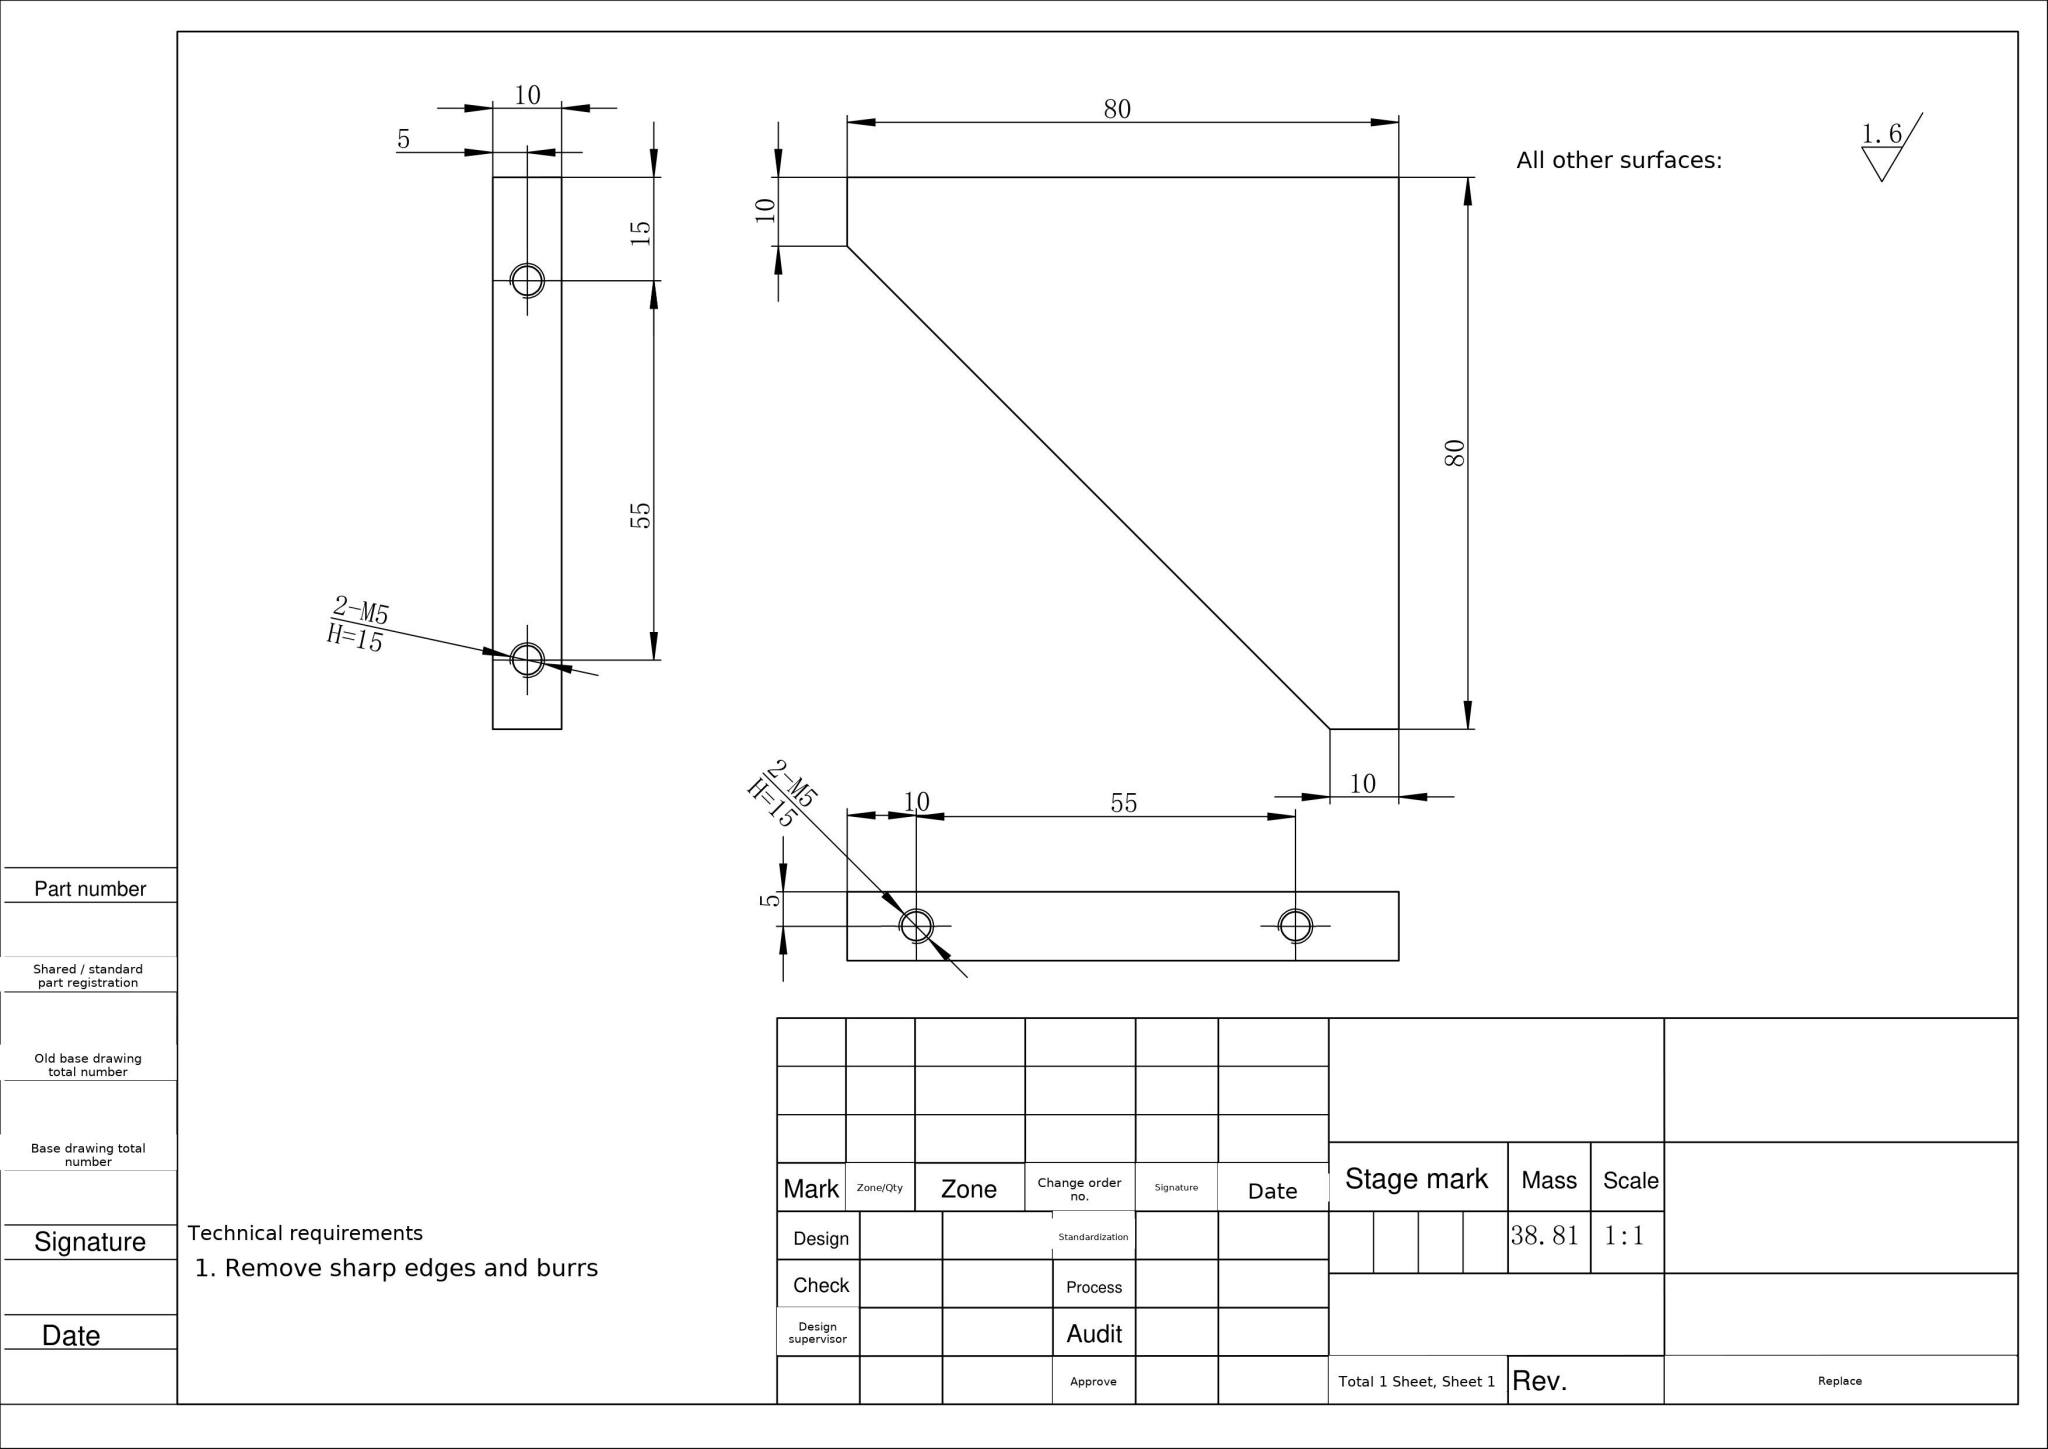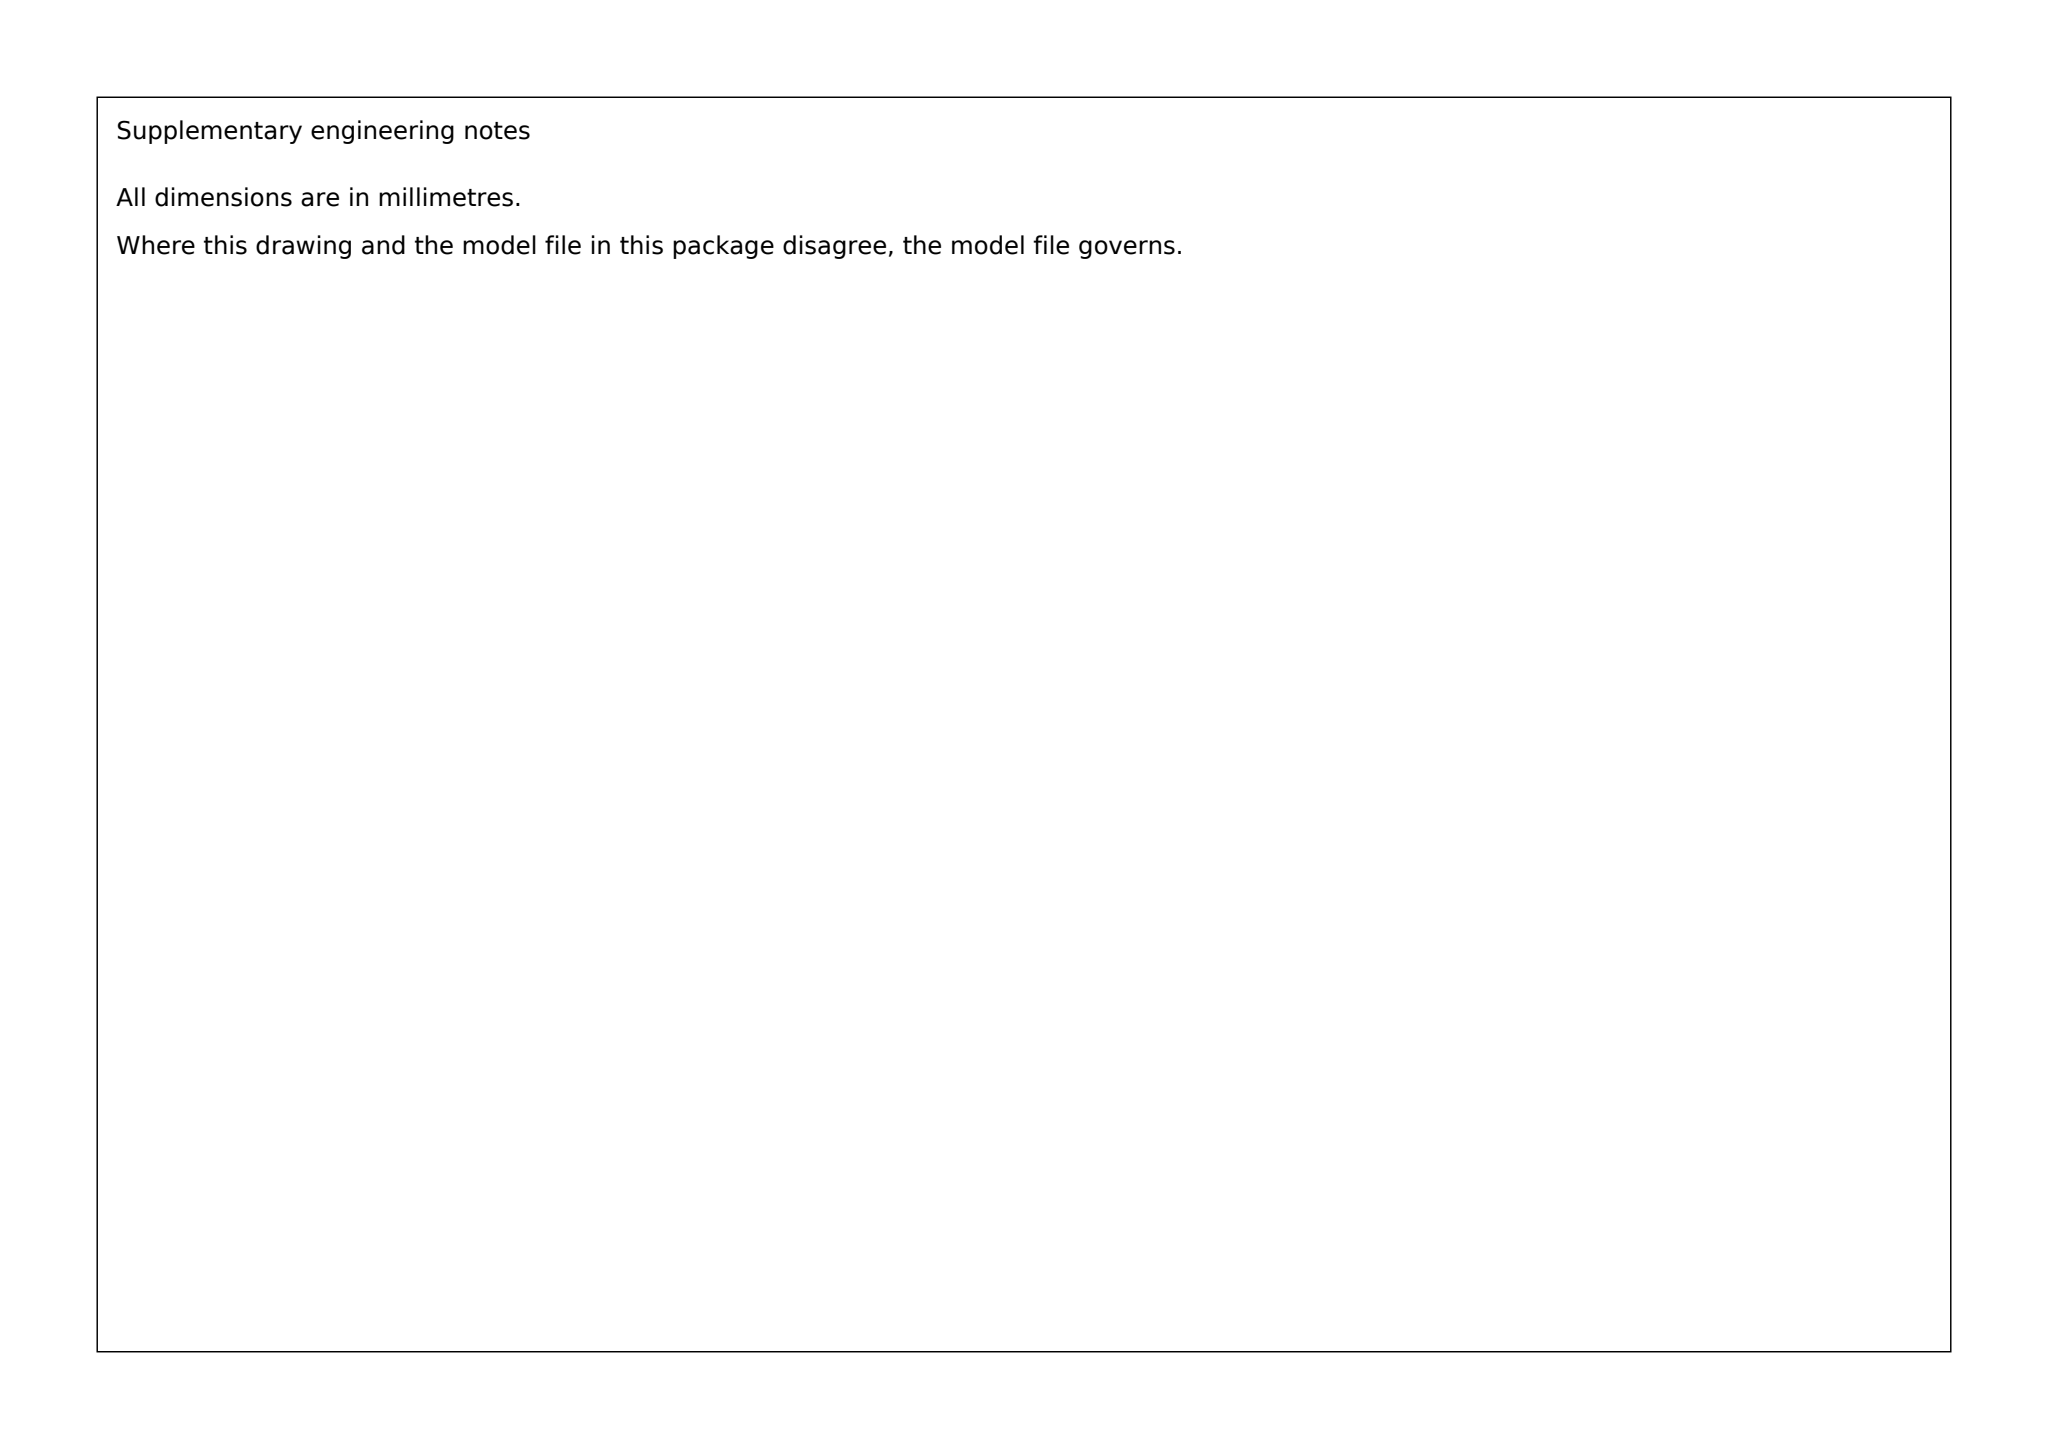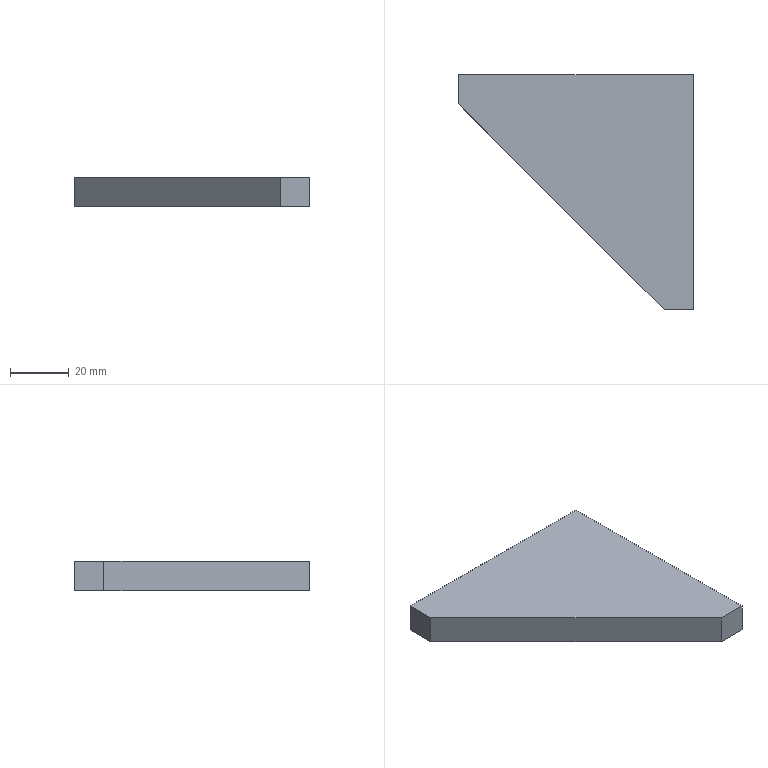Part | SolidWorks | mm | 1 solid | 23 faces | box 80 x 80 x 10 mm | volume 38812 mm3 | cylinder 8 | cone 8 | plane 7 | commonest cylinder face diameters 4.2 x8
build123d program:
from build123d import *

# Parameters (mm, degrees)
BOSS_EXTRUDE1_DEPTH   = 10
M5_TAPPED_HOLE1_D     = 4.2
M5_TAPPED_HOLE1_DEPTH = 12
M5_TAPPED_HOLE1_TIP   = 1.262
M5_TAPPED_HOLE2_D     = 4.2
M5_TAPPED_HOLE2_DEPTH = 12
M5_TAPPED_HOLE2_TIP   = 1.262


with BuildPart() as part:
    # Sketch1 → Boss-Extrude1 (new body)
    with BuildSketch(Plane.XY):
        Polygon((571.382, 0), (571.382, -80), (561.382, -80), (491.382, -10), (491.382, 0), align=None)
    extrude(amount=-BOSS_EXTRUDE1_DEPTH)

    # M5 Tapped Hole1
    with Locations(Plane(origin=(0, 0, 0), x_dir=(1, 0, 0), z_dir=(0, 1, 0))):
        with Locations((556.382, 5), (501.382, 5)):
            Hole(M5_TAPPED_HOLE1_D / 2, depth=M5_TAPPED_HOLE1_DEPTH)
            with Locations((0, 0, -(M5_TAPPED_HOLE1_DEPTH + M5_TAPPED_HOLE1_TIP / 2))):  # 118° drill point
                Cone(0, M5_TAPPED_HOLE1_D / 2, M5_TAPPED_HOLE1_TIP, mode=Mode.SUBTRACT)

    # M5 Tapped Hole2
    with Locations(Plane(origin=(571.382, 0, 0), x_dir=(0, 0, -1), z_dir=(1, 0, 0))):
        with Locations((5, -70), (5, -15)):
            Hole(M5_TAPPED_HOLE2_D / 2, depth=M5_TAPPED_HOLE2_DEPTH)
            with Locations((0, 0, -(M5_TAPPED_HOLE2_DEPTH + M5_TAPPED_HOLE2_TIP / 2))):  # 118° drill point
                Cone(0, M5_TAPPED_HOLE2_D / 2, M5_TAPPED_HOLE2_TIP, mode=Mode.SUBTRACT)


solid = part.part
STEP:
#1=CARTESIAN_POINT('',(559.382,-15.,-2.9));
#2=VERTEX_POINT('',#1);
#3=CARTESIAN_POINT('',(559.382,-15.,-7.1));
#4=VERTEX_POINT('',#3);
#5=CARTESIAN_POINT('',(559.382,-15.,-5.));
#6=DIRECTION('',(1.,0.,0.));
#7=DIRECTION('',(0.,0.,-1.));
#8=AXIS2_PLACEMENT_3D('',#5,#6,#7);
#9=CIRCLE('',#8,2.1);
#10=EDGE_CURVE('',#2,#4,#9,.T.);
#11=ORIENTED_EDGE('',*,*,#10,.F.);
#12=CARTESIAN_POINT('',(571.382,-15.,-2.9));
#13=VERTEX_POINT('',#12);
#14=CARTESIAN_POINT('',(571.382,-15.,-2.9));
#15=DIRECTION('',(1.,0.,0.));
#16=VECTOR('',#15,1000.);
#17=LINE('',#14,#16);
#18=EDGE_CURVE('',#2,#13,#17,.T.);
#19=ORIENTED_EDGE('',*,*,#18,.T.);
#20=CARTESIAN_POINT('',(571.382,-15.,-7.1));
#21=VERTEX_POINT('',#20);
#22=CARTESIAN_POINT('',(571.382,-15.,-5.));
#23=DIRECTION('',(1.,0.,0.));
#24=DIRECTION('',(0.,0.,-1.));
#25=AXIS2_PLACEMENT_3D('',#22,#23,#24);
#26=CIRCLE('',#25,2.1);
#27=EDGE_CURVE('',#13,#21,#26,.T.);
#28=ORIENTED_EDGE('',*,*,#27,.T.);
#29=CARTESIAN_POINT('',(571.382,-15.,-7.1));
#30=DIRECTION('',(1.,0.,0.));
#31=VECTOR('',#30,1000.);
#32=LINE('',#29,#31);
#33=EDGE_CURVE('',#4,#21,#32,.T.);
#34=ORIENTED_EDGE('',*,*,#33,.F.);
#35=EDGE_LOOP('',(#11,#19,#28,#34));
#36=FACE_OUTER_BOUND('',#35,.T.);
#37=CARTESIAN_POINT('',(571.382,-15.,-5.));
#38=DIRECTION('',(1.,0.,0.));
#39=DIRECTION('',(0.,0.,-1.));
#40=AXIS2_PLACEMENT_3D('',#37,#38,#39);
#41=CYLINDRICAL_SURFACE('',#40,2.1);
#42=ADVANCED_FACE('',(#36),#41,.F.);
#43=CARTESIAN_POINT('',(558.12,-15.,-5.));
#44=VERTEX_POINT('',#43);
#45=CARTESIAN_POINT('',(559.382,-15.,-7.1));
#46=DIRECTION('',(0.515,0.,-0.8572));
#47=VECTOR('',#46,1000.);
#48=LINE('',#45,#47);
#49=EDGE_CURVE('',#44,#4,#48,.T.);
#50=ORIENTED_EDGE('',*,*,#49,.F.);
#51=CARTESIAN_POINT('',(559.382,-15.,-2.9));
#52=DIRECTION('',(0.515,0.,0.8572));
#53=VECTOR('',#52,1000.);
#54=LINE('',#51,#53);
#55=EDGE_CURVE('',#44,#2,#54,.T.);
#56=ORIENTED_EDGE('',*,*,#55,.T.);
#57=ORIENTED_EDGE('',*,*,#10,.T.);
#58=EDGE_LOOP('',(#50,#56,#57));
#59=FACE_OUTER_BOUND('',#58,.T.);
#60=CARTESIAN_POINT('',(559.382,-15.,-5.));
#61=DIRECTION('',(1.,0.,0.));
#62=DIRECTION('',(0.,0.,-1.));
#63=AXIS2_PLACEMENT_3D('',#60,#61,#62);
#64=CONICAL_SURFACE('',#63,2.1,1.03);
#65=ADVANCED_FACE('',(#59),#64,.F.);
#66=CARTESIAN_POINT('',(559.382,-70.,-2.9));
#67=VERTEX_POINT('',#66);
#68=CARTESIAN_POINT('',(559.382,-70.,-7.1));
#69=VERTEX_POINT('',#68);
#70=CARTESIAN_POINT('',(559.382,-70.,-5.));
#71=DIRECTION('',(1.,0.,0.));
#72=DIRECTION('',(0.,0.,-1.));
#73=AXIS2_PLACEMENT_3D('',#70,#71,#72);
#74=CIRCLE('',#73,2.1);
#75=EDGE_CURVE('',#67,#69,#74,.T.);
#76=ORIENTED_EDGE('',*,*,#75,.F.);
#77=CARTESIAN_POINT('',(571.382,-70.,-2.9));
#78=VERTEX_POINT('',#77);
#79=CARTESIAN_POINT('',(571.382,-70.,-2.9));
#80=DIRECTION('',(1.,0.,0.));
#81=VECTOR('',#80,1000.);
#82=LINE('',#79,#81);
#83=EDGE_CURVE('',#67,#78,#82,.T.);
#84=ORIENTED_EDGE('',*,*,#83,.T.);
#85=CARTESIAN_POINT('',(571.382,-70.,-7.1));
#86=VERTEX_POINT('',#85);
#87=CARTESIAN_POINT('',(571.382,-70.,-5.));
#88=DIRECTION('',(1.,0.,0.));
#89=DIRECTION('',(0.,0.,-1.));
#90=AXIS2_PLACEMENT_3D('',#87,#88,#89);
#91=CIRCLE('',#90,2.1);
#92=EDGE_CURVE('',#78,#86,#91,.T.);
#93=ORIENTED_EDGE('',*,*,#92,.T.);
#94=CARTESIAN_POINT('',(571.382,-70.,-7.1));
#95=DIRECTION('',(1.,0.,0.));
#96=VECTOR('',#95,1000.);
#97=LINE('',#94,#96);
#98=EDGE_CURVE('',#69,#86,#97,.T.);
#99=ORIENTED_EDGE('',*,*,#98,.F.);
#100=EDGE_LOOP('',(#76,#84,#93,#99));
#101=FACE_OUTER_BOUND('',#100,.T.);
#102=CARTESIAN_POINT('',(571.382,-70.,-5.));
#103=DIRECTION('',(1.,0.,0.));
#104=DIRECTION('',(0.,0.,-1.));
#105=AXIS2_PLACEMENT_3D('',#102,#103,#104);
#106=CYLINDRICAL_SURFACE('',#105,2.1);
#107=ADVANCED_FACE('',(#101),#106,.F.);
#108=CARTESIAN_POINT('',(558.12,-70.,-5.));
#109=VERTEX_POINT('',#108);
#110=CARTESIAN_POINT('',(559.382,-70.,-7.1));
#111=DIRECTION('',(0.515,0.,-0.8572));
#112=VECTOR('',#111,1000.);
#113=LINE('',#110,#112);
#114=EDGE_CURVE('',#109,#69,#113,.T.);
#115=ORIENTED_EDGE('',*,*,#114,.F.);
#116=CARTESIAN_POINT('',(559.382,-70.,-2.9));
#117=DIRECTION('',(0.515,0.,0.8572));
#118=VECTOR('',#117,1000.);
#119=LINE('',#116,#118);
#120=EDGE_CURVE('',#109,#67,#119,.T.);
#121=ORIENTED_EDGE('',*,*,#120,.T.);
#122=ORIENTED_EDGE('',*,*,#75,.T.);
#123=EDGE_LOOP('',(#115,#121,#122));
#124=FACE_OUTER_BOUND('',#123,.T.);
#125=CARTESIAN_POINT('',(559.382,-70.,-5.));
#126=DIRECTION('',(1.,0.,0.));
#127=DIRECTION('',(0.,0.,-1.));
#128=AXIS2_PLACEMENT_3D('',#125,#126,#127);
#129=CONICAL_SURFACE('',#128,2.1,1.03);
#130=ADVANCED_FACE('',(#124),#129,.F.);
#131=CARTESIAN_POINT('',(501.382,-12.,-7.1));
#132=VERTEX_POINT('',#131);
#133=CARTESIAN_POINT('',(501.382,-12.,-2.9));
#134=VERTEX_POINT('',#133);
#135=CARTESIAN_POINT('',(501.382,-12.,-5.));
#136=DIRECTION('',(0.,1.,0.));
#137=DIRECTION('',(0.,0.,1.));
#138=AXIS2_PLACEMENT_3D('',#135,#136,#137);
#139=CIRCLE('',#138,2.1);
#140=EDGE_CURVE('',#132,#134,#139,.T.);
#141=ORIENTED_EDGE('',*,*,#140,.F.);
#142=CARTESIAN_POINT('',(501.382,0.,-7.1));
#143=VERTEX_POINT('',#142);
#144=CARTESIAN_POINT('',(501.382,-0.,-7.1));
#145=DIRECTION('',(0.,1.,0.));
#146=VECTOR('',#145,1000.);
#147=LINE('',#144,#146);
#148=EDGE_CURVE('',#132,#143,#147,.T.);
#149=ORIENTED_EDGE('',*,*,#148,.T.);
#150=CARTESIAN_POINT('',(501.382,0.,-2.9));
#151=VERTEX_POINT('',#150);
#152=CARTESIAN_POINT('',(501.382,0.,-5.));
#153=DIRECTION('',(0.,1.,0.));
#154=DIRECTION('',(0.,0.,1.));
#155=AXIS2_PLACEMENT_3D('',#152,#153,#154);
#156=CIRCLE('',#155,2.1);
#157=EDGE_CURVE('',#143,#151,#156,.T.);
#158=ORIENTED_EDGE('',*,*,#157,.T.);
#159=CARTESIAN_POINT('',(501.382,-0.,-2.9));
#160=DIRECTION('',(0.,1.,0.));
#161=VECTOR('',#160,1000.);
#162=LINE('',#159,#161);
#163=EDGE_CURVE('',#134,#151,#162,.T.);
#164=ORIENTED_EDGE('',*,*,#163,.F.);
#165=EDGE_LOOP('',(#141,#149,#158,#164));
#166=FACE_OUTER_BOUND('',#165,.T.);
#167=CARTESIAN_POINT('',(501.382,-0.,-5.));
#168=DIRECTION('',(0.,1.,0.));
#169=DIRECTION('',(0.,0.,1.));
#170=AXIS2_PLACEMENT_3D('',#167,#168,#169);
#171=CYLINDRICAL_SURFACE('',#170,2.1);
#172=ADVANCED_FACE('',(#166),#171,.F.);
#173=CARTESIAN_POINT('',(501.382,-13.262,-5.));
#174=VERTEX_POINT('',#173);
#175=CARTESIAN_POINT('',(501.382,-12.,-2.9));
#176=DIRECTION('',(0.,0.515,0.8572));
#177=VECTOR('',#176,1000.);
#178=LINE('',#175,#177);
#179=EDGE_CURVE('',#174,#134,#178,.T.);
#180=ORIENTED_EDGE('',*,*,#179,.F.);
#181=CARTESIAN_POINT('',(501.382,-12.,-7.1));
#182=DIRECTION('',(0.,0.515,-0.8572));
#183=VECTOR('',#182,1000.);
#184=LINE('',#181,#183);
#185=EDGE_CURVE('',#174,#132,#184,.T.);
#186=ORIENTED_EDGE('',*,*,#185,.T.);
#187=ORIENTED_EDGE('',*,*,#140,.T.);
#188=EDGE_LOOP('',(#180,#186,#187));
#189=FACE_OUTER_BOUND('',#188,.T.);
#190=CARTESIAN_POINT('',(501.382,-12.,-5.));
#191=DIRECTION('',(0.,1.,0.));
#192=DIRECTION('',(0.,0.,1.));
#193=AXIS2_PLACEMENT_3D('',#190,#191,#192);
#194=CONICAL_SURFACE('',#193,2.1,1.03);
#195=ADVANCED_FACE('',(#189),#194,.F.);
#196=CARTESIAN_POINT('',(556.382,-12.,-7.1));
#197=VERTEX_POINT('',#196);
#198=CARTESIAN_POINT('',(556.382,-12.,-2.9));
#199=VERTEX_POINT('',#198);
#200=CARTESIAN_POINT('',(556.382,-12.,-5.));
#201=DIRECTION('',(0.,1.,0.));
#202=DIRECTION('',(0.,0.,1.));
#203=AXIS2_PLACEMENT_3D('',#200,#201,#202);
#204=CIRCLE('',#203,2.1);
#205=EDGE_CURVE('',#197,#199,#204,.T.);
#206=ORIENTED_EDGE('',*,*,#205,.F.);
#207=CARTESIAN_POINT('',(556.382,0.,-7.1));
#208=VERTEX_POINT('',#207);
#209=CARTESIAN_POINT('',(556.382,-0.,-7.1));
#210=DIRECTION('',(0.,1.,0.));
#211=VECTOR('',#210,1000.);
#212=LINE('',#209,#211);
#213=EDGE_CURVE('',#197,#208,#212,.T.);
#214=ORIENTED_EDGE('',*,*,#213,.T.);
#215=CARTESIAN_POINT('',(556.382,0.,-2.9));
#216=VERTEX_POINT('',#215);
#217=CARTESIAN_POINT('',(556.382,0.,-5.));
#218=DIRECTION('',(0.,1.,0.));
#219=DIRECTION('',(0.,0.,1.));
#220=AXIS2_PLACEMENT_3D('',#217,#218,#219);
#221=CIRCLE('',#220,2.1);
#222=EDGE_CURVE('',#208,#216,#221,.T.);
#223=ORIENTED_EDGE('',*,*,#222,.T.);
#224=CARTESIAN_POINT('',(556.382,-0.,-2.9));
#225=DIRECTION('',(0.,1.,0.));
#226=VECTOR('',#225,1000.);
#227=LINE('',#224,#226);
#228=EDGE_CURVE('',#199,#216,#227,.T.);
#229=ORIENTED_EDGE('',*,*,#228,.F.);
#230=EDGE_LOOP('',(#206,#214,#223,#229));
#231=FACE_OUTER_BOUND('',#230,.T.);
#232=CARTESIAN_POINT('',(556.382,-0.,-5.));
#233=DIRECTION('',(0.,1.,0.));
#234=DIRECTION('',(0.,0.,1.));
#235=AXIS2_PLACEMENT_3D('',#232,#233,#234);
#236=CYLINDRICAL_SURFACE('',#235,2.1);
#237=ADVANCED_FACE('',(#231),#236,.F.);
#238=CARTESIAN_POINT('',(556.382,-13.262,-5.));
#239=VERTEX_POINT('',#238);
#240=CARTESIAN_POINT('',(556.382,-12.,-2.9));
#241=DIRECTION('',(0.,0.515,0.8572));
#242=VECTOR('',#241,1000.);
#243=LINE('',#240,#242);
#244=EDGE_CURVE('',#239,#199,#243,.T.);
#245=ORIENTED_EDGE('',*,*,#244,.F.);
#246=CARTESIAN_POINT('',(556.382,-12.,-7.1));
#247=DIRECTION('',(0.,0.515,-0.8572));
#248=VECTOR('',#247,1000.);
#249=LINE('',#246,#248);
#250=EDGE_CURVE('',#239,#197,#249,.T.);
#251=ORIENTED_EDGE('',*,*,#250,.T.);
#252=ORIENTED_EDGE('',*,*,#205,.T.);
#253=EDGE_LOOP('',(#245,#251,#252));
#254=FACE_OUTER_BOUND('',#253,.T.);
#255=CARTESIAN_POINT('',(556.382,-12.,-5.));
#256=DIRECTION('',(0.,1.,0.));
#257=DIRECTION('',(0.,0.,1.));
#258=AXIS2_PLACEMENT_3D('',#255,#256,#257);
#259=CONICAL_SURFACE('',#258,2.1,1.03);
#260=ADVANCED_FACE('',(#254),#259,.F.);
#261=CARTESIAN_POINT('',(501.382,0.,-5.));
#262=DIRECTION('',(0.,1.,0.));
#263=DIRECTION('',(0.,0.,1.));
#264=AXIS2_PLACEMENT_3D('',#261,#262,#263);
#265=CIRCLE('',#264,2.1);
#266=EDGE_CURVE('',#151,#143,#265,.T.);
#267=ORIENTED_EDGE('',*,*,#266,.F.);
#268=ORIENTED_EDGE('',*,*,#157,.F.);
#269=EDGE_LOOP('',(#267,#268));
#270=FACE_BOUND('',#269,.T.);
#271=CARTESIAN_POINT('',(556.382,0.,-5.));
#272=DIRECTION('',(0.,1.,0.));
#273=DIRECTION('',(0.,0.,1.));
#274=AXIS2_PLACEMENT_3D('',#271,#272,#273);
#275=CIRCLE('',#274,2.1);
#276=EDGE_CURVE('',#216,#208,#275,.T.);
#277=ORIENTED_EDGE('',*,*,#276,.F.);
#278=ORIENTED_EDGE('',*,*,#222,.F.);
#279=EDGE_LOOP('',(#277,#278));
#280=FACE_BOUND('',#279,.T.);
#281=CARTESIAN_POINT('',(571.382,0.,0.));
#282=VERTEX_POINT('',#281);
#283=CARTESIAN_POINT('',(491.382,0.,0.));
#284=VERTEX_POINT('',#283);
#285=CARTESIAN_POINT('',(491.382,0.,0.));
#286=DIRECTION('',(-1.,0.,0.));
#287=VECTOR('',#286,1000.);
#288=LINE('',#285,#287);
#289=EDGE_CURVE('',#282,#284,#288,.T.);
#290=ORIENTED_EDGE('',*,*,#289,.F.);
#291=CARTESIAN_POINT('',(571.382,0.,-10.));
#292=VERTEX_POINT('',#291);
#293=CARTESIAN_POINT('',(571.382,0.,-10.));
#294=DIRECTION('',(0.,0.,1.));
#295=VECTOR('',#294,1000.);
#296=LINE('',#293,#295);
#297=EDGE_CURVE('',#292,#282,#296,.T.);
#298=ORIENTED_EDGE('',*,*,#297,.F.);
#299=CARTESIAN_POINT('',(491.382,0.,-10.));
#300=VERTEX_POINT('',#299);
#301=CARTESIAN_POINT('',(491.382,0.,-10.));
#302=DIRECTION('',(-1.,0.,0.));
#303=VECTOR('',#302,1000.);
#304=LINE('',#301,#303);
#305=EDGE_CURVE('',#292,#300,#304,.T.);
#306=ORIENTED_EDGE('',*,*,#305,.T.);
#307=CARTESIAN_POINT('',(491.382,0.,-10.));
#308=DIRECTION('',(0.,0.,1.));
#309=VECTOR('',#308,1000.);
#310=LINE('',#307,#309);
#311=EDGE_CURVE('',#300,#284,#310,.T.);
#312=ORIENTED_EDGE('',*,*,#311,.T.);
#313=EDGE_LOOP('',(#290,#298,#306,#312));
#314=FACE_OUTER_BOUND('',#313,.T.);
#315=CARTESIAN_POINT('',(491.382,0.,-10.));
#316=DIRECTION('',(0.,1.,0.));
#317=DIRECTION('',(-1.,0.,0.));
#318=AXIS2_PLACEMENT_3D('',#315,#316,#317);
#319=PLANE('',#318);
#320=ADVANCED_FACE('',(#270,#280,#314),#319,.T.);
#321=CARTESIAN_POINT('',(571.382,-15.,-5.));
#322=DIRECTION('',(1.,0.,0.));
#323=DIRECTION('',(0.,0.,-1.));
#324=AXIS2_PLACEMENT_3D('',#321,#322,#323);
#325=CIRCLE('',#324,2.1);
#326=EDGE_CURVE('',#21,#13,#325,.T.);
#327=ORIENTED_EDGE('',*,*,#326,.F.);
#328=ORIENTED_EDGE('',*,*,#27,.F.);
#329=EDGE_LOOP('',(#327,#328));
#330=FACE_BOUND('',#329,.T.);
#331=CARTESIAN_POINT('',(571.382,-70.,-5.));
#332=DIRECTION('',(1.,0.,0.));
#333=DIRECTION('',(0.,0.,-1.));
#334=AXIS2_PLACEMENT_3D('',#331,#332,#333);
#335=CIRCLE('',#334,2.1);
#336=EDGE_CURVE('',#86,#78,#335,.T.);
#337=ORIENTED_EDGE('',*,*,#336,.F.);
#338=ORIENTED_EDGE('',*,*,#92,.F.);
#339=EDGE_LOOP('',(#337,#338));
#340=FACE_BOUND('',#339,.T.);
#341=CARTESIAN_POINT('',(571.382,-80.,0.));
#342=VERTEX_POINT('',#341);
#343=CARTESIAN_POINT('',(571.382,0.,0.));
#344=DIRECTION('',(0.,1.,0.));
#345=VECTOR('',#344,1000.);
#346=LINE('',#343,#345);
#347=EDGE_CURVE('',#342,#282,#346,.T.);
#348=ORIENTED_EDGE('',*,*,#347,.F.);
#349=CARTESIAN_POINT('',(571.382,-80.,-10.));
#350=VERTEX_POINT('',#349);
#351=CARTESIAN_POINT('',(571.382,-80.,-10.));
#352=DIRECTION('',(0.,0.,1.));
#353=VECTOR('',#352,1000.);
#354=LINE('',#351,#353);
#355=EDGE_CURVE('',#350,#342,#354,.T.);
#356=ORIENTED_EDGE('',*,*,#355,.F.);
#357=CARTESIAN_POINT('',(571.382,0.,-10.));
#358=DIRECTION('',(0.,1.,0.));
#359=VECTOR('',#358,1000.);
#360=LINE('',#357,#359);
#361=EDGE_CURVE('',#350,#292,#360,.T.);
#362=ORIENTED_EDGE('',*,*,#361,.T.);
#363=ORIENTED_EDGE('',*,*,#297,.T.);
#364=EDGE_LOOP('',(#348,#356,#362,#363));
#365=FACE_OUTER_BOUND('',#364,.T.);
#366=CARTESIAN_POINT('',(571.382,0.,-10.));
#367=DIRECTION('',(1.,0.,0.));
#368=DIRECTION('',(0.,0.,-1.));
#369=AXIS2_PLACEMENT_3D('',#366,#367,#368);
#370=PLANE('',#369);
#371=ADVANCED_FACE('',(#330,#340,#365),#370,.T.);
#372=CARTESIAN_POINT('',(561.382,-80.,0.));
#373=VERTEX_POINT('',#372);
#374=CARTESIAN_POINT('',(561.382,-80.,0.));
#375=DIRECTION('',(1.,0.,0.));
#376=VECTOR('',#375,1000.);
#377=LINE('',#374,#376);
#378=EDGE_CURVE('',#373,#342,#377,.T.);
#379=ORIENTED_EDGE('',*,*,#378,.F.);
#380=CARTESIAN_POINT('',(561.382,-80.,-10.));
#381=VERTEX_POINT('',#380);
#382=CARTESIAN_POINT('',(561.382,-80.,-10.));
#383=DIRECTION('',(0.,0.,1.));
#384=VECTOR('',#383,1000.);
#385=LINE('',#382,#384);
#386=EDGE_CURVE('',#381,#373,#385,.T.);
#387=ORIENTED_EDGE('',*,*,#386,.F.);
#388=CARTESIAN_POINT('',(561.382,-80.,-10.));
#389=DIRECTION('',(1.,0.,0.));
#390=VECTOR('',#389,1000.);
#391=LINE('',#388,#390);
#392=EDGE_CURVE('',#381,#350,#391,.T.);
#393=ORIENTED_EDGE('',*,*,#392,.T.);
#394=ORIENTED_EDGE('',*,*,#355,.T.);
#395=EDGE_LOOP('',(#379,#387,#393,#394));
#396=FACE_OUTER_BOUND('',#395,.T.);
#397=CARTESIAN_POINT('',(561.382,-80.,-10.));
#398=DIRECTION('',(0.,-1.,0.));
#399=DIRECTION('',(0.,0.,-1.));
#400=AXIS2_PLACEMENT_3D('',#397,#398,#399);
#401=PLANE('',#400);
#402=ADVANCED_FACE('',(#396),#401,.T.);
#403=CARTESIAN_POINT('',(491.382,-10.,0.));
#404=VERTEX_POINT('',#403);
#405=CARTESIAN_POINT('',(491.382,-10.,0.));
#406=DIRECTION('',(0.7071,-0.7071,0.));
#407=VECTOR('',#406,1000.);
#408=LINE('',#405,#407);
#409=EDGE_CURVE('',#404,#373,#408,.T.);
#410=ORIENTED_EDGE('',*,*,#409,.F.);
#411=CARTESIAN_POINT('',(491.382,-10.,-10.));
#412=VERTEX_POINT('',#411);
#413=CARTESIAN_POINT('',(491.382,-10.,-10.));
#414=DIRECTION('',(0.,0.,1.));
#415=VECTOR('',#414,1000.);
#416=LINE('',#413,#415);
#417=EDGE_CURVE('',#412,#404,#416,.T.);
#418=ORIENTED_EDGE('',*,*,#417,.F.);
#419=CARTESIAN_POINT('',(491.382,-10.,-10.));
#420=DIRECTION('',(0.7071,-0.7071,0.));
#421=VECTOR('',#420,1000.);
#422=LINE('',#419,#421);
#423=EDGE_CURVE('',#412,#381,#422,.T.);
#424=ORIENTED_EDGE('',*,*,#423,.T.);
#425=ORIENTED_EDGE('',*,*,#386,.T.);
#426=EDGE_LOOP('',(#410,#418,#424,#425));
#427=FACE_OUTER_BOUND('',#426,.T.);
#428=CARTESIAN_POINT('',(491.382,-10.,-10.));
#429=DIRECTION('',(-0.7071,-0.7071,0.));
#430=DIRECTION('',(0.7071,-0.7071,0.));
#431=AXIS2_PLACEMENT_3D('',#428,#429,#430);
#432=PLANE('',#431);
#433=ADVANCED_FACE('',(#427),#432,.T.);
#434=CARTESIAN_POINT('',(491.382,0.,0.));
#435=DIRECTION('',(0.,-1.,0.));
#436=VECTOR('',#435,1000.);
#437=LINE('',#434,#436);
#438=EDGE_CURVE('',#284,#404,#437,.T.);
#439=ORIENTED_EDGE('',*,*,#438,.F.);
#440=ORIENTED_EDGE('',*,*,#311,.F.);
#441=CARTESIAN_POINT('',(491.382,0.,-10.));
#442=DIRECTION('',(0.,-1.,0.));
#443=VECTOR('',#442,1000.);
#444=LINE('',#441,#443);
#445=EDGE_CURVE('',#300,#412,#444,.T.);
#446=ORIENTED_EDGE('',*,*,#445,.T.);
#447=ORIENTED_EDGE('',*,*,#417,.T.);
#448=EDGE_LOOP('',(#439,#440,#446,#447));
#449=FACE_OUTER_BOUND('',#448,.T.);
#450=CARTESIAN_POINT('',(491.382,0.,-10.));
#451=DIRECTION('',(-1.,0.,0.));
#452=DIRECTION('',(0.,0.,1.));
#453=AXIS2_PLACEMENT_3D('',#450,#451,#452);
#454=PLANE('',#453);
#455=ADVANCED_FACE('',(#449),#454,.T.);
#456=ORIENTED_EDGE('',*,*,#305,.F.);
#457=ORIENTED_EDGE('',*,*,#361,.F.);
#458=ORIENTED_EDGE('',*,*,#392,.F.);
#459=ORIENTED_EDGE('',*,*,#423,.F.);
#460=ORIENTED_EDGE('',*,*,#445,.F.);
#461=EDGE_LOOP('',(#456,#457,#458,#459,#460));
#462=FACE_OUTER_BOUND('',#461,.T.);
#463=CARTESIAN_POINT('',(0.,0.,-10.));
#464=DIRECTION('',(0.,0.,-1.));
#465=DIRECTION('',(-1.,0.,0.));
#466=AXIS2_PLACEMENT_3D('',#463,#464,#465);
#467=PLANE('',#466);
#468=ADVANCED_FACE('',(#462),#467,.T.);
#469=ORIENTED_EDGE('',*,*,#289,.T.);
#470=ORIENTED_EDGE('',*,*,#438,.T.);
#471=ORIENTED_EDGE('',*,*,#409,.T.);
#472=ORIENTED_EDGE('',*,*,#378,.T.);
#473=ORIENTED_EDGE('',*,*,#347,.T.);
#474=EDGE_LOOP('',(#469,#470,#471,#472,#473));
#475=FACE_OUTER_BOUND('',#474,.T.);
#476=CARTESIAN_POINT('',(0.,0.,0.));
#477=DIRECTION('',(0.,0.,-1.));
#478=DIRECTION('',(-1.,0.,0.));
#479=AXIS2_PLACEMENT_3D('',#476,#477,#478);
#480=PLANE('',#479);
#481=ADVANCED_FACE('',(#475),#480,.F.);
#482=ORIENTED_EDGE('',*,*,#250,.F.);
#483=ORIENTED_EDGE('',*,*,#244,.T.);
#484=CARTESIAN_POINT('',(556.382,-12.,-5.));
#485=DIRECTION('',(0.,1.,0.));
#486=DIRECTION('',(0.,0.,1.));
#487=AXIS2_PLACEMENT_3D('',#484,#485,#486);
#488=CIRCLE('',#487,2.1);
#489=EDGE_CURVE('',#199,#197,#488,.T.);
#490=ORIENTED_EDGE('',*,*,#489,.T.);
#491=EDGE_LOOP('',(#482,#483,#490));
#492=FACE_OUTER_BOUND('',#491,.T.);
#493=CARTESIAN_POINT('',(556.382,-12.,-5.));
#494=DIRECTION('',(0.,1.,0.));
#495=DIRECTION('',(0.,0.,1.));
#496=AXIS2_PLACEMENT_3D('',#493,#494,#495);
#497=CONICAL_SURFACE('',#496,2.1,1.03);
#498=ADVANCED_FACE('',(#492),#497,.F.);
#499=ORIENTED_EDGE('',*,*,#213,.F.);
#500=ORIENTED_EDGE('',*,*,#489,.F.);
#501=ORIENTED_EDGE('',*,*,#228,.T.);
#502=ORIENTED_EDGE('',*,*,#276,.T.);
#503=EDGE_LOOP('',(#499,#500,#501,#502));
#504=FACE_OUTER_BOUND('',#503,.T.);
#505=CARTESIAN_POINT('',(556.382,-0.,-5.));
#506=DIRECTION('',(0.,1.,0.));
#507=DIRECTION('',(0.,0.,1.));
#508=AXIS2_PLACEMENT_3D('',#505,#506,#507);
#509=CYLINDRICAL_SURFACE('',#508,2.1);
#510=ADVANCED_FACE('',(#504),#509,.F.);
#511=ORIENTED_EDGE('',*,*,#185,.F.);
#512=ORIENTED_EDGE('',*,*,#179,.T.);
#513=CARTESIAN_POINT('',(501.382,-12.,-5.));
#514=DIRECTION('',(0.,1.,0.));
#515=DIRECTION('',(0.,0.,1.));
#516=AXIS2_PLACEMENT_3D('',#513,#514,#515);
#517=CIRCLE('',#516,2.1);
#518=EDGE_CURVE('',#134,#132,#517,.T.);
#519=ORIENTED_EDGE('',*,*,#518,.T.);
#520=EDGE_LOOP('',(#511,#512,#519));
#521=FACE_OUTER_BOUND('',#520,.T.);
#522=CARTESIAN_POINT('',(501.382,-12.,-5.));
#523=DIRECTION('',(0.,1.,0.));
#524=DIRECTION('',(0.,0.,1.));
#525=AXIS2_PLACEMENT_3D('',#522,#523,#524);
#526=CONICAL_SURFACE('',#525,2.1,1.03);
#527=ADVANCED_FACE('',(#521),#526,.F.);
#528=ORIENTED_EDGE('',*,*,#148,.F.);
#529=ORIENTED_EDGE('',*,*,#518,.F.);
#530=ORIENTED_EDGE('',*,*,#163,.T.);
#531=ORIENTED_EDGE('',*,*,#266,.T.);
#532=EDGE_LOOP('',(#528,#529,#530,#531));
#533=FACE_OUTER_BOUND('',#532,.T.);
#534=CARTESIAN_POINT('',(501.382,-0.,-5.));
#535=DIRECTION('',(0.,1.,0.));
#536=DIRECTION('',(0.,0.,1.));
#537=AXIS2_PLACEMENT_3D('',#534,#535,#536);
#538=CYLINDRICAL_SURFACE('',#537,2.1);
#539=ADVANCED_FACE('',(#533),#538,.F.);
#540=ORIENTED_EDGE('',*,*,#120,.F.);
#541=ORIENTED_EDGE('',*,*,#114,.T.);
#542=CARTESIAN_POINT('',(559.382,-70.,-5.));
#543=DIRECTION('',(1.,0.,0.));
#544=DIRECTION('',(0.,0.,-1.));
#545=AXIS2_PLACEMENT_3D('',#542,#543,#544);
#546=CIRCLE('',#545,2.1);
#547=EDGE_CURVE('',#69,#67,#546,.T.);
#548=ORIENTED_EDGE('',*,*,#547,.T.);
#549=EDGE_LOOP('',(#540,#541,#548));
#550=FACE_OUTER_BOUND('',#549,.T.);
#551=CARTESIAN_POINT('',(559.382,-70.,-5.));
#552=DIRECTION('',(1.,0.,0.));
#553=DIRECTION('',(0.,0.,-1.));
#554=AXIS2_PLACEMENT_3D('',#551,#552,#553);
#555=CONICAL_SURFACE('',#554,2.1,1.03);
#556=ADVANCED_FACE('',(#550),#555,.F.);
#557=ORIENTED_EDGE('',*,*,#83,.F.);
#558=ORIENTED_EDGE('',*,*,#547,.F.);
#559=ORIENTED_EDGE('',*,*,#98,.T.);
#560=ORIENTED_EDGE('',*,*,#336,.T.);
#561=EDGE_LOOP('',(#557,#558,#559,#560));
#562=FACE_OUTER_BOUND('',#561,.T.);
#563=CARTESIAN_POINT('',(571.382,-70.,-5.));
#564=DIRECTION('',(1.,0.,0.));
#565=DIRECTION('',(0.,0.,-1.));
#566=AXIS2_PLACEMENT_3D('',#563,#564,#565);
#567=CYLINDRICAL_SURFACE('',#566,2.1);
#568=ADVANCED_FACE('',(#562),#567,.F.);
#569=ORIENTED_EDGE('',*,*,#55,.F.);
#570=ORIENTED_EDGE('',*,*,#49,.T.);
#571=CARTESIAN_POINT('',(559.382,-15.,-5.));
#572=DIRECTION('',(1.,0.,0.));
#573=DIRECTION('',(0.,0.,-1.));
#574=AXIS2_PLACEMENT_3D('',#571,#572,#573);
#575=CIRCLE('',#574,2.1);
#576=EDGE_CURVE('',#4,#2,#575,.T.);
#577=ORIENTED_EDGE('',*,*,#576,.T.);
#578=EDGE_LOOP('',(#569,#570,#577));
#579=FACE_OUTER_BOUND('',#578,.T.);
#580=CARTESIAN_POINT('',(559.382,-15.,-5.));
#581=DIRECTION('',(1.,0.,0.));
#582=DIRECTION('',(0.,0.,-1.));
#583=AXIS2_PLACEMENT_3D('',#580,#581,#582);
#584=CONICAL_SURFACE('',#583,2.1,1.03);
#585=ADVANCED_FACE('',(#579),#584,.F.);
#586=ORIENTED_EDGE('',*,*,#18,.F.);
#587=ORIENTED_EDGE('',*,*,#576,.F.);
#588=ORIENTED_EDGE('',*,*,#33,.T.);
#589=ORIENTED_EDGE('',*,*,#326,.T.);
#590=EDGE_LOOP('',(#586,#587,#588,#589));
#591=FACE_OUTER_BOUND('',#590,.T.);
#592=CARTESIAN_POINT('',(571.382,-15.,-5.));
#593=DIRECTION('',(1.,0.,0.));
#594=DIRECTION('',(0.,0.,-1.));
#595=AXIS2_PLACEMENT_3D('',#592,#593,#594);
#596=CYLINDRICAL_SURFACE('',#595,2.1);
#597=ADVANCED_FACE('',(#591),#596,.F.);
#598=CLOSED_SHELL('',(#42,#65,#107,#130,#172,#195,#237,#260,#320,#371,#402,#433,#455,#468,#481,#498,#510,#527,#539,#556,#568,#585,#597));
#599=MANIFOLD_SOLID_BREP('',#598);
#600=CARTESIAN_POINT('',(0.,0.,0.));
#601=DIRECTION('',(0.,0.,1.));
#602=DIRECTION('',(1.,0.,0.));
#603=AXIS2_PLACEMENT_3D('',#600,#601,#602);
#604=(LENGTH_UNIT()NAMED_UNIT(*)SI_UNIT(.MILLI.,.METRE.));
#605=UNCERTAINTY_MEASURE_WITH_UNIT(LENGTH_MEASURE(0.00001),#604,'','');
#606=(NAMED_UNIT(*)PLANE_ANGLE_UNIT()SI_UNIT($,.RADIAN.));
#607=(NAMED_UNIT(*)SI_UNIT($,.STERADIAN.)SOLID_ANGLE_UNIT());
#608=(GEOMETRIC_REPRESENTATION_CONTEXT(3)GLOBAL_UNCERTAINTY_ASSIGNED_CONTEXT((#605))GLOBAL_UNIT_ASSIGNED_CONTEXT((#604,#606,#607))REPRESENTATION_CONTEXT('',''));
#609=ADVANCED_BREP_SHAPE_REPRESENTATION('',(#599,#603),#608);